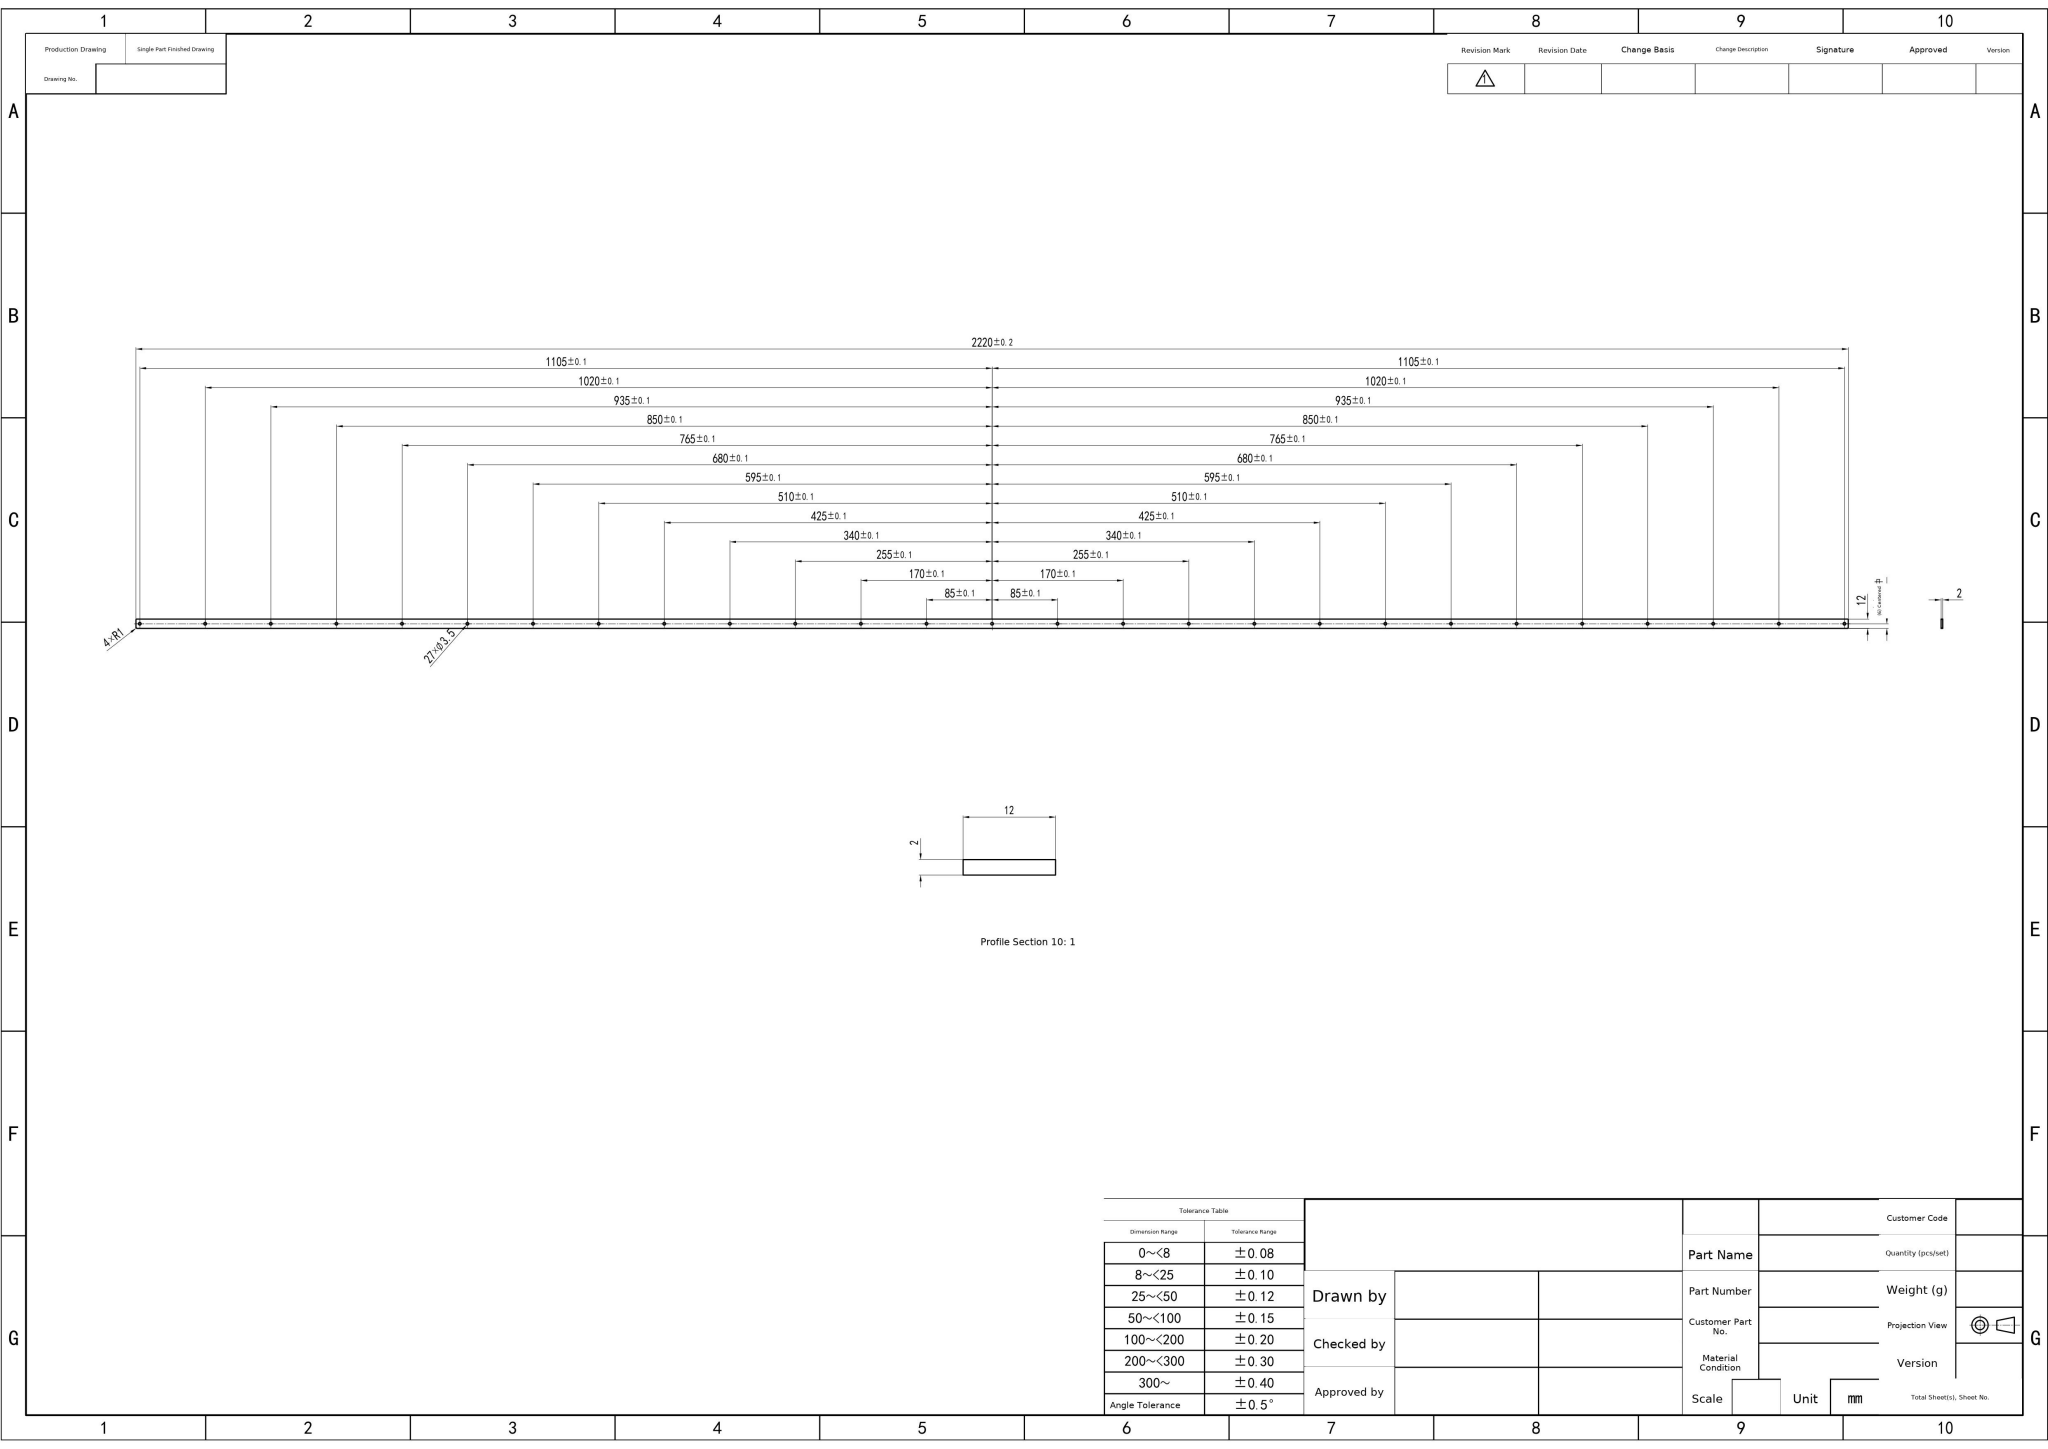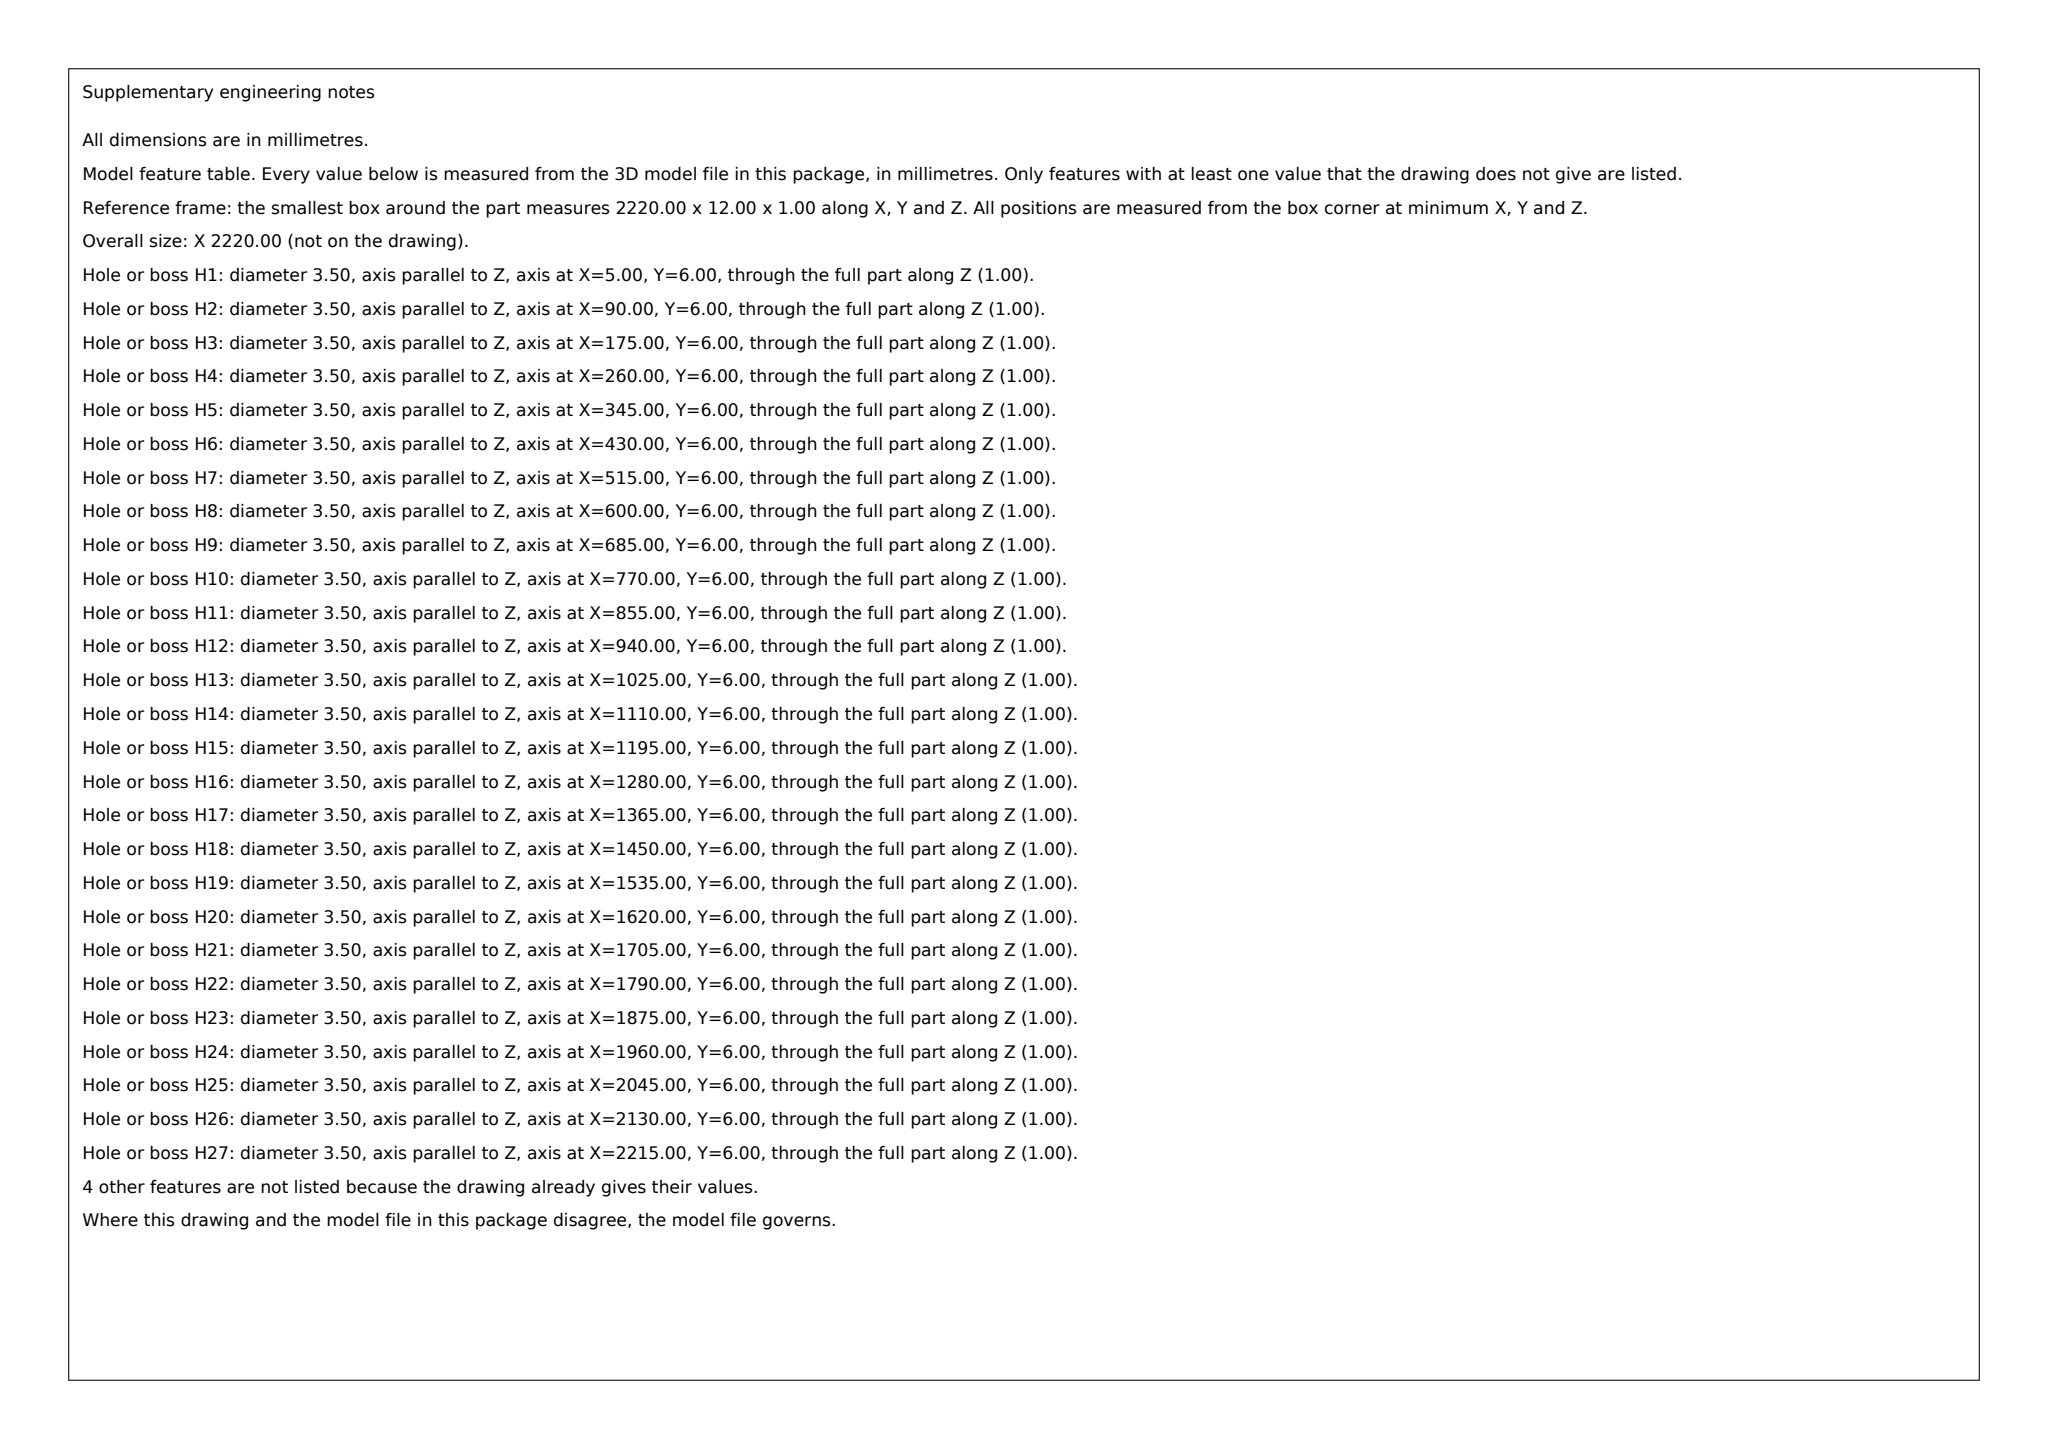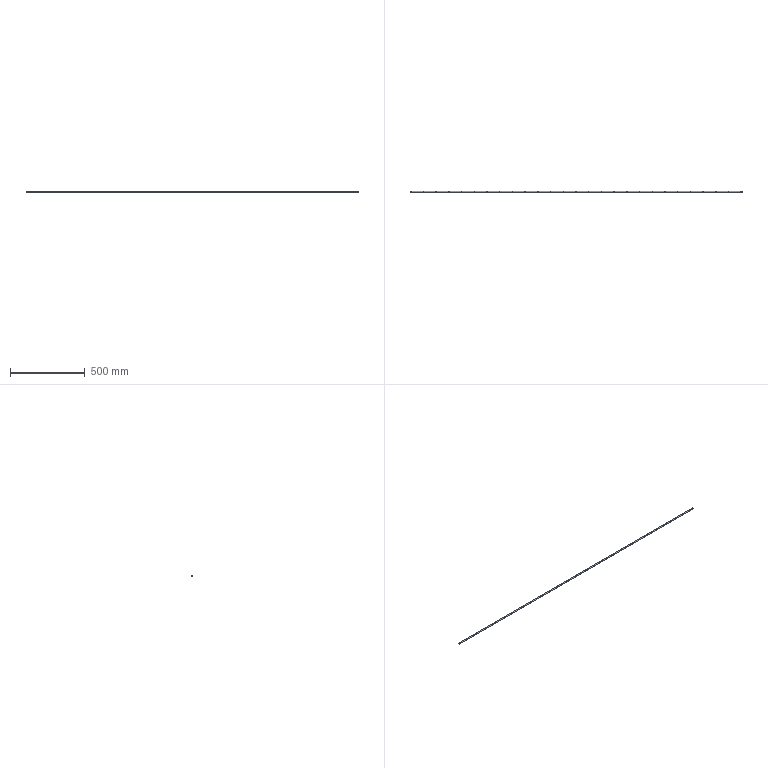Part | SolidWorks | mm | 1 solid | 64 faces | box 2220 x 12 x 1 mm | volume 26379 mm3 | cylinder 58 | plane 6 | commonest cylinder face diameters 3.5 x54 2 x4